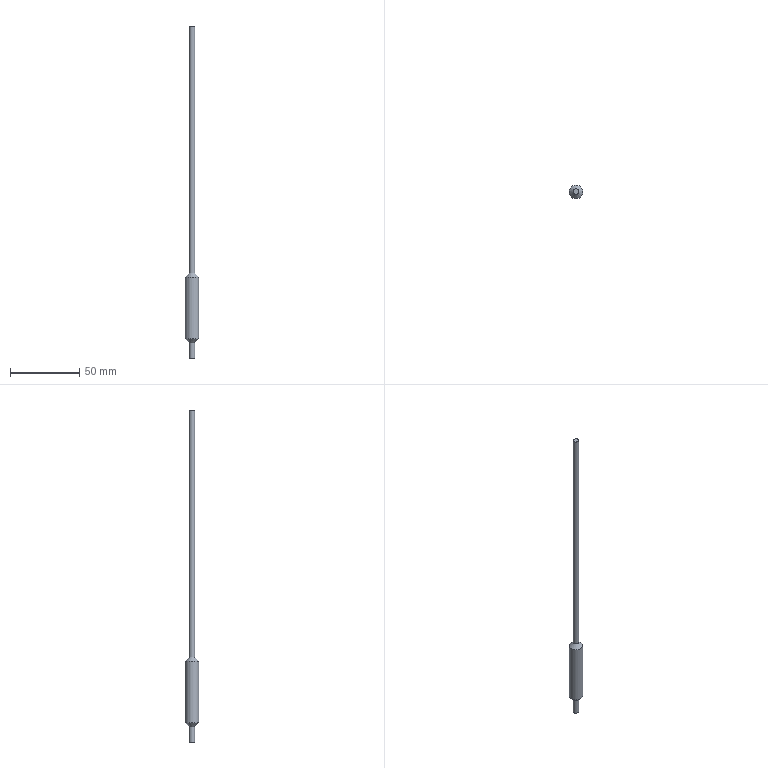Component | NX | MANDREL | 1 solid | 7 faces | box 10 x 10 x 239 mm | volume 6076 mm3 | cylinder 3 | plane 2 | cone 2 | commonest cylinder face diameters 4 x2 10 x1
STEP:
#1=CARTESIAN_POINT('',(0.,0.,0.));
#2=DIRECTION('',(0.,0.,1.));
#3=DIRECTION('',(1.,0.,0.));
#4=AXIS2_PLACEMENT_3D('',#1,#2,#3);
#5=CARTESIAN_POINT('',(-146.777,2.,63.4));
#6=VERTEX_POINT('',#5);
#7=CARTESIAN_POINT('',(-146.777,0.,63.4));
#8=DIRECTION('',(0.,0.,-1.));
#9=DIRECTION('',(0.,1.,0.));
#10=AXIS2_PLACEMENT_3D('',#7,#8,#9);
#11=CIRCLE('',#10,2.);
#12=CARTESIAN_POINT('',(-146.777,0.,63.4));
#13=DIRECTION('',(0.,0.,-1.));
#14=DIRECTION('',(0.,1.,0.));
#15=AXIS2_PLACEMENT_3D('',#12,#13,#14);
#16=PLANE('',#15);
#17=CARTESIAN_POINT('',(0.,0.));
#18=DIRECTION('',(1.,0.));
#19=AXIS2_PLACEMENT_2D('',#17,#18);
#20=CIRCLE('',#19,2.);
#21=(GEOMETRIC_REPRESENTATION_CONTEXT(2)PARAMETRIC_REPRESENTATION_CONTEXT()REPRESENTATION_CONTEXT('',''));
#22=DEFINITIONAL_REPRESENTATION('',(#20),#21);
#23=PCURVE('',#16,#22);
#24=CARTESIAN_POINT('',(-146.777,0.,63.4));
#25=DIRECTION('',(0.,0.,-1.));
#26=DIRECTION('',(0.,1.,0.));
#27=AXIS2_PLACEMENT_3D('',#24,#25,#26);
#28=CYLINDRICAL_SURFACE('',#27,2.);
#29=CARTESIAN_POINT('',(0.,0.));
#30=DIRECTION('',(1.,0.));
#31=VECTOR('',#30,1.);
#32=LINE('',#29,#31);
#33=(GEOMETRIC_REPRESENTATION_CONTEXT(2)PARAMETRIC_REPRESENTATION_CONTEXT()REPRESENTATION_CONTEXT('',''));
#34=DEFINITIONAL_REPRESENTATION('',(#32),#33);
#35=PCURVE('',#28,#34);
#36=SURFACE_CURVE('',#11,(#23,#35),.PCURVE_S1.);
#37=EDGE_CURVE('',#6,#6,#36,.T.);
#38=ORIENTED_EDGE('',*,*,#37,.T.);
#39=EDGE_LOOP('',(#38));
#40=FACE_BOUND('',#39,.T.);
#41=ADVANCED_FACE('',(#40),#16,.T.);
#42=CARTESIAN_POINT('',(-146.777,2.,74.4));
#43=VERTEX_POINT('',#42);
#44=CARTESIAN_POINT('',(-146.777,0.,74.4));
#45=DIRECTION('',(0.,0.,-1.));
#46=DIRECTION('',(0.,1.,0.));
#47=AXIS2_PLACEMENT_3D('',#44,#45,#46);
#48=CIRCLE('',#47,2.);
#49=CARTESIAN_POINT('',(0.,-11.));
#50=DIRECTION('',(1.,0.));
#51=VECTOR('',#50,1.);
#52=LINE('',#49,#51);
#53=(GEOMETRIC_REPRESENTATION_CONTEXT(2)PARAMETRIC_REPRESENTATION_CONTEXT()REPRESENTATION_CONTEXT('',''));
#54=DEFINITIONAL_REPRESENTATION('',(#52),#53);
#55=PCURVE('',#28,#54);
#56=CARTESIAN_POINT('',(-146.777,0.,74.4));
#57=DIRECTION('',(0.,0.,1.));
#58=DIRECTION('',(0.,-1.,0.));
#59=AXIS2_PLACEMENT_3D('',#56,#57,#58);
#60=CONICAL_SURFACE('',#59,2.,0.7854);
#61=CARTESIAN_POINT('',(9.425,0.));
#62=DIRECTION('',(-1.,0.));
#63=VECTOR('',#62,1.);
#64=LINE('',#61,#63);
#65=(GEOMETRIC_REPRESENTATION_CONTEXT(2)PARAMETRIC_REPRESENTATION_CONTEXT()REPRESENTATION_CONTEXT('',''));
#66=DEFINITIONAL_REPRESENTATION('',(#64),#65);
#67=PCURVE('',#60,#66);
#68=SURFACE_CURVE('',#48,(#55,#67),.PCURVE_S1.);
#69=EDGE_CURVE('',#43,#43,#68,.T.);
#70=ORIENTED_EDGE('',*,*,#69,.T.);
#71=CARTESIAN_POINT('',(-146.777,2.,74.4));
#72=CARTESIAN_POINT('',(-146.777,2.,63.4));
#73=B_SPLINE_CURVE_WITH_KNOTS('',1,(#71,#72),.UNSPECIFIED.,.F.,.F.,(2,2),(-11.,0.),.PIECEWISE_BEZIER_KNOTS.);
#74=CARTESIAN_POINT('',(6.283,0.));
#75=DIRECTION('',(0.,1.));
#76=VECTOR('',#75,1.);
#77=LINE('',#74,#76);
#78=(GEOMETRIC_REPRESENTATION_CONTEXT(2)PARAMETRIC_REPRESENTATION_CONTEXT()REPRESENTATION_CONTEXT('',''));
#79=DEFINITIONAL_REPRESENTATION('',(#77),#78);
#80=PCURVE('',#28,#79);
#81=CARTESIAN_POINT('',(0.,0.));
#82=DIRECTION('',(0.,1.));
#83=VECTOR('',#82,1.);
#84=LINE('',#81,#83);
#85=(GEOMETRIC_REPRESENTATION_CONTEXT(2)PARAMETRIC_REPRESENTATION_CONTEXT()REPRESENTATION_CONTEXT('',''));
#86=DEFINITIONAL_REPRESENTATION('',(#84),#85);
#87=PCURVE('',#28,#86);
#88=SEAM_CURVE('',#73,(#80,#87),.PCURVE_S1.);
#89=EDGE_CURVE('',#43,#6,#88,.T.);
#90=ORIENTED_EDGE('',*,*,#89,.T.);
#91=ORIENTED_EDGE('',*,*,#37,.F.);
#92=ORIENTED_EDGE('',*,*,#89,.F.);
#93=EDGE_LOOP('',(#70,#90,#91,#92));
#94=FACE_BOUND('',#93,.T.);
#95=ADVANCED_FACE('',(#94),#28,.T.);
#96=CARTESIAN_POINT('',(-146.777,5.,77.4));
#97=VERTEX_POINT('',#96);
#98=CARTESIAN_POINT('',(-146.777,0.,77.4));
#99=DIRECTION('',(0.,0.,-1.));
#100=DIRECTION('',(0.,1.,0.));
#101=AXIS2_PLACEMENT_3D('',#98,#99,#100);
#102=CIRCLE('',#101,5.);
#103=CARTESIAN_POINT('',(9.425,3.));
#104=DIRECTION('',(-1.,0.));
#105=VECTOR('',#104,1.);
#106=LINE('',#103,#105);
#107=(GEOMETRIC_REPRESENTATION_CONTEXT(2)PARAMETRIC_REPRESENTATION_CONTEXT()REPRESENTATION_CONTEXT('',''));
#108=DEFINITIONAL_REPRESENTATION('',(#106),#107);
#109=PCURVE('',#60,#108);
#110=CARTESIAN_POINT('',(-146.777,0.,63.4));
#111=DIRECTION('',(0.,0.,-1.));
#112=DIRECTION('',(0.,1.,0.));
#113=AXIS2_PLACEMENT_3D('',#110,#111,#112);
#114=CYLINDRICAL_SURFACE('',#113,5.);
#115=CARTESIAN_POINT('',(0.,-14.));
#116=DIRECTION('',(1.,0.));
#117=VECTOR('',#116,1.);
#118=LINE('',#115,#117);
#119=(GEOMETRIC_REPRESENTATION_CONTEXT(2)PARAMETRIC_REPRESENTATION_CONTEXT()REPRESENTATION_CONTEXT('',''));
#120=DEFINITIONAL_REPRESENTATION('',(#118),#119);
#121=PCURVE('',#114,#120);
#122=SURFACE_CURVE('',#102,(#109,#121),.PCURVE_S1.);
#123=EDGE_CURVE('',#97,#97,#122,.T.);
#124=ORIENTED_EDGE('',*,*,#123,.T.);
#125=CARTESIAN_POINT('',(-146.777,2.,74.4));
#126=CARTESIAN_POINT('',(-146.777,5.,77.4));
#127=B_SPLINE_CURVE_WITH_KNOTS('',1,(#125,#126),.UNSPECIFIED.,.F.,.F.,(2,2),(0.,4.243),.PIECEWISE_BEZIER_KNOTS.);
#128=CARTESIAN_POINT('',(3.142,0.));
#129=DIRECTION('',(0.,1.));
#130=VECTOR('',#129,1.);
#131=LINE('',#128,#130);
#132=(GEOMETRIC_REPRESENTATION_CONTEXT(2)PARAMETRIC_REPRESENTATION_CONTEXT()REPRESENTATION_CONTEXT('',''));
#133=DEFINITIONAL_REPRESENTATION('',(#131),#132);
#134=PCURVE('',#60,#133);
#135=CARTESIAN_POINT('',(9.425,0.));
#136=DIRECTION('',(0.,1.));
#137=VECTOR('',#136,1.);
#138=LINE('',#135,#137);
#139=(GEOMETRIC_REPRESENTATION_CONTEXT(2)PARAMETRIC_REPRESENTATION_CONTEXT()REPRESENTATION_CONTEXT('',''));
#140=DEFINITIONAL_REPRESENTATION('',(#138),#139);
#141=PCURVE('',#60,#140);
#142=SEAM_CURVE('',#127,(#134,#141),.PCURVE_S1.);
#143=EDGE_CURVE('',#43,#97,#142,.T.);
#144=ORIENTED_EDGE('',*,*,#143,.F.);
#145=ORIENTED_EDGE('',*,*,#69,.F.);
#146=ORIENTED_EDGE('',*,*,#143,.T.);
#147=EDGE_LOOP('',(#124,#144,#145,#146));
#148=FACE_BOUND('',#147,.T.);
#149=ADVANCED_FACE('',(#148),#60,.T.);
#150=CARTESIAN_POINT('',(-146.777,5.,121.4));
#151=VERTEX_POINT('',#150);
#152=CARTESIAN_POINT('',(-146.777,0.,121.4));
#153=DIRECTION('',(0.,0.,-1.));
#154=DIRECTION('',(0.,1.,0.));
#155=AXIS2_PLACEMENT_3D('',#152,#153,#154);
#156=CIRCLE('',#155,5.);
#157=CARTESIAN_POINT('',(0.,-58.));
#158=DIRECTION('',(1.,0.));
#159=VECTOR('',#158,1.);
#160=LINE('',#157,#159);
#161=(GEOMETRIC_REPRESENTATION_CONTEXT(2)PARAMETRIC_REPRESENTATION_CONTEXT()REPRESENTATION_CONTEXT('',''));
#162=DEFINITIONAL_REPRESENTATION('',(#160),#161);
#163=PCURVE('',#114,#162);
#164=CARTESIAN_POINT('',(-146.777,0.,121.4));
#165=DIRECTION('',(0.,0.,-1.));
#166=DIRECTION('',(0.,1.,0.));
#167=AXIS2_PLACEMENT_3D('',#164,#165,#166);
#168=CONICAL_SURFACE('',#167,5.,0.7854);
#169=CARTESIAN_POINT('',(0.,0.));
#170=DIRECTION('',(1.,0.));
#171=VECTOR('',#170,1.);
#172=LINE('',#169,#171);
#173=(GEOMETRIC_REPRESENTATION_CONTEXT(2)PARAMETRIC_REPRESENTATION_CONTEXT()REPRESENTATION_CONTEXT('',''));
#174=DEFINITIONAL_REPRESENTATION('',(#172),#173);
#175=PCURVE('',#168,#174);
#176=SURFACE_CURVE('',#156,(#163,#175),.PCURVE_S1.);
#177=EDGE_CURVE('',#151,#151,#176,.T.);
#178=ORIENTED_EDGE('',*,*,#177,.T.);
#179=CARTESIAN_POINT('',(-146.777,5.,121.4));
#180=CARTESIAN_POINT('',(-146.777,5.,77.4));
#181=B_SPLINE_CURVE_WITH_KNOTS('',1,(#179,#180),.UNSPECIFIED.,.F.,.F.,(2,2),(-58.,-14.),.PIECEWISE_BEZIER_KNOTS.);
#182=CARTESIAN_POINT('',(6.283,0.));
#183=DIRECTION('',(0.,1.));
#184=VECTOR('',#183,1.);
#185=LINE('',#182,#184);
#186=(GEOMETRIC_REPRESENTATION_CONTEXT(2)PARAMETRIC_REPRESENTATION_CONTEXT()REPRESENTATION_CONTEXT('',''));
#187=DEFINITIONAL_REPRESENTATION('',(#185),#186);
#188=PCURVE('',#114,#187);
#189=CARTESIAN_POINT('',(0.,0.));
#190=DIRECTION('',(0.,1.));
#191=VECTOR('',#190,1.);
#192=LINE('',#189,#191);
#193=(GEOMETRIC_REPRESENTATION_CONTEXT(2)PARAMETRIC_REPRESENTATION_CONTEXT()REPRESENTATION_CONTEXT('',''));
#194=DEFINITIONAL_REPRESENTATION('',(#192),#193);
#195=PCURVE('',#114,#194);
#196=SEAM_CURVE('',#181,(#188,#195),.PCURVE_S1.);
#197=EDGE_CURVE('',#151,#97,#196,.T.);
#198=ORIENTED_EDGE('',*,*,#197,.T.);
#199=ORIENTED_EDGE('',*,*,#123,.F.);
#200=ORIENTED_EDGE('',*,*,#197,.F.);
#201=EDGE_LOOP('',(#178,#198,#199,#200));
#202=FACE_BOUND('',#201,.T.);
#203=ADVANCED_FACE('',(#202),#114,.T.);
#204=CARTESIAN_POINT('',(-146.777,2.,124.4));
#205=VERTEX_POINT('',#204);
#206=CARTESIAN_POINT('',(-146.777,0.,124.4));
#207=DIRECTION('',(0.,0.,-1.));
#208=DIRECTION('',(0.,1.,0.));
#209=AXIS2_PLACEMENT_3D('',#206,#207,#208);
#210=CIRCLE('',#209,2.);
#211=CARTESIAN_POINT('',(0.,-3.));
#212=DIRECTION('',(1.,0.));
#213=VECTOR('',#212,1.);
#214=LINE('',#211,#213);
#215=(GEOMETRIC_REPRESENTATION_CONTEXT(2)PARAMETRIC_REPRESENTATION_CONTEXT()REPRESENTATION_CONTEXT('',''));
#216=DEFINITIONAL_REPRESENTATION('',(#214),#215);
#217=PCURVE('',#168,#216);
#218=CARTESIAN_POINT('',(-146.777,0.,63.4));
#219=DIRECTION('',(0.,0.,-1.));
#220=DIRECTION('',(0.,1.,0.));
#221=AXIS2_PLACEMENT_3D('',#218,#219,#220);
#222=CYLINDRICAL_SURFACE('',#221,2.);
#223=CARTESIAN_POINT('',(0.,-61.));
#224=DIRECTION('',(1.,0.));
#225=VECTOR('',#224,1.);
#226=LINE('',#223,#225);
#227=(GEOMETRIC_REPRESENTATION_CONTEXT(2)PARAMETRIC_REPRESENTATION_CONTEXT()REPRESENTATION_CONTEXT('',''));
#228=DEFINITIONAL_REPRESENTATION('',(#226),#227);
#229=PCURVE('',#222,#228);
#230=SURFACE_CURVE('',#210,(#217,#229),.PCURVE_S1.);
#231=EDGE_CURVE('',#205,#205,#230,.T.);
#232=ORIENTED_EDGE('',*,*,#231,.T.);
#233=CARTESIAN_POINT('',(-146.777,2.,124.4));
#234=CARTESIAN_POINT('',(-146.777,5.,121.4));
#235=B_SPLINE_CURVE_WITH_KNOTS('',1,(#233,#234),.UNSPECIFIED.,.F.,.F.,(2,2),(-4.243,0.),.PIECEWISE_BEZIER_KNOTS.);
#236=CARTESIAN_POINT('',(6.283,0.));
#237=DIRECTION('',(0.,1.));
#238=VECTOR('',#237,1.);
#239=LINE('',#236,#238);
#240=(GEOMETRIC_REPRESENTATION_CONTEXT(2)PARAMETRIC_REPRESENTATION_CONTEXT()REPRESENTATION_CONTEXT('',''));
#241=DEFINITIONAL_REPRESENTATION('',(#239),#240);
#242=PCURVE('',#168,#241);
#243=CARTESIAN_POINT('',(0.,0.));
#244=DIRECTION('',(0.,1.));
#245=VECTOR('',#244,1.);
#246=LINE('',#243,#245);
#247=(GEOMETRIC_REPRESENTATION_CONTEXT(2)PARAMETRIC_REPRESENTATION_CONTEXT()REPRESENTATION_CONTEXT('',''));
#248=DEFINITIONAL_REPRESENTATION('',(#246),#247);
#249=PCURVE('',#168,#248);
#250=SEAM_CURVE('',#235,(#242,#249),.PCURVE_S1.);
#251=EDGE_CURVE('',#205,#151,#250,.T.);
#252=ORIENTED_EDGE('',*,*,#251,.T.);
#253=ORIENTED_EDGE('',*,*,#177,.F.);
#254=ORIENTED_EDGE('',*,*,#251,.F.);
#255=EDGE_LOOP('',(#232,#252,#253,#254));
#256=FACE_BOUND('',#255,.T.);
#257=ADVANCED_FACE('',(#256),#168,.T.);
#258=CARTESIAN_POINT('',(-146.777,2.,302.4));
#259=VERTEX_POINT('',#258);
#260=CARTESIAN_POINT('',(-146.777,0.,302.4));
#261=DIRECTION('',(0.,0.,-1.));
#262=DIRECTION('',(0.,1.,0.));
#263=AXIS2_PLACEMENT_3D('',#260,#261,#262);
#264=CIRCLE('',#263,2.);
#265=CARTESIAN_POINT('',(0.,-239.));
#266=DIRECTION('',(1.,0.));
#267=VECTOR('',#266,1.);
#268=LINE('',#265,#267);
#269=(GEOMETRIC_REPRESENTATION_CONTEXT(2)PARAMETRIC_REPRESENTATION_CONTEXT()REPRESENTATION_CONTEXT('',''));
#270=DEFINITIONAL_REPRESENTATION('',(#268),#269);
#271=PCURVE('',#222,#270);
#272=CARTESIAN_POINT('',(-144.777,0.,302.4));
#273=DIRECTION('',(0.,0.,1.));
#274=DIRECTION('',(0.,-1.,0.));
#275=AXIS2_PLACEMENT_3D('',#272,#273,#274);
#276=PLANE('',#275);
#277=CARTESIAN_POINT('',(-2.,-2.));
#278=CARTESIAN_POINT('',(-2.,1.464));
#279=CARTESIAN_POINT('',(1.,-0.2679));
#280=CARTESIAN_POINT('',(4.,-2.));
#281=CARTESIAN_POINT('',(1.,-3.732));
#282=CARTESIAN_POINT('',(-2.,-5.464));
#283=CARTESIAN_POINT('',(-2.,-2.));
#284=(BOUNDED_CURVE()B_SPLINE_CURVE(2,(#277,#278,#279,#280,#281,#282,#283),.UNSPECIFIED.,.T.,.F.)B_SPLINE_CURVE_WITH_KNOTS((1,2,2,2,2,1),(-2.094,0.,2.094,4.189,6.283,8.378),.UNSPECIFIED.)CURVE()GEOMETRIC_REPRESENTATION_ITEM()RATIONAL_B_SPLINE_CURVE((1.,0.5,1.,0.5,1.,0.5,1.))REPRESENTATION_ITEM(''));
#285=(GEOMETRIC_REPRESENTATION_CONTEXT(2)PARAMETRIC_REPRESENTATION_CONTEXT()REPRESENTATION_CONTEXT('',''));
#286=DEFINITIONAL_REPRESENTATION('',(#284),#285);
#287=PCURVE('',#276,#286);
#288=SURFACE_CURVE('',#264,(#271,#287),.PCURVE_S1.);
#289=EDGE_CURVE('',#259,#259,#288,.T.);
#290=ORIENTED_EDGE('',*,*,#289,.T.);
#291=CARTESIAN_POINT('',(-146.777,2.,302.4));
#292=CARTESIAN_POINT('',(-146.777,2.,124.4));
#293=B_SPLINE_CURVE_WITH_KNOTS('',1,(#291,#292),.UNSPECIFIED.,.F.,.F.,(2,2),(-239.,-61.),.PIECEWISE_BEZIER_KNOTS.);
#294=CARTESIAN_POINT('',(6.283,0.));
#295=DIRECTION('',(0.,1.));
#296=VECTOR('',#295,1.);
#297=LINE('',#294,#296);
#298=(GEOMETRIC_REPRESENTATION_CONTEXT(2)PARAMETRIC_REPRESENTATION_CONTEXT()REPRESENTATION_CONTEXT('',''));
#299=DEFINITIONAL_REPRESENTATION('',(#297),#298);
#300=PCURVE('',#222,#299);
#301=CARTESIAN_POINT('',(0.,0.));
#302=DIRECTION('',(0.,1.));
#303=VECTOR('',#302,1.);
#304=LINE('',#301,#303);
#305=(GEOMETRIC_REPRESENTATION_CONTEXT(2)PARAMETRIC_REPRESENTATION_CONTEXT()REPRESENTATION_CONTEXT('',''));
#306=DEFINITIONAL_REPRESENTATION('',(#304),#305);
#307=PCURVE('',#222,#306);
#308=SEAM_CURVE('',#293,(#300,#307),.PCURVE_S1.);
#309=EDGE_CURVE('',#259,#205,#308,.T.);
#310=ORIENTED_EDGE('',*,*,#309,.T.);
#311=ORIENTED_EDGE('',*,*,#231,.F.);
#312=ORIENTED_EDGE('',*,*,#309,.F.);
#313=EDGE_LOOP('',(#290,#310,#311,#312));
#314=FACE_BOUND('',#313,.T.);
#315=ADVANCED_FACE('',(#314),#222,.T.);
#316=ORIENTED_EDGE('',*,*,#289,.F.);
#317=EDGE_LOOP('',(#316));
#318=FACE_BOUND('',#317,.T.);
#319=ADVANCED_FACE('',(#318),#276,.T.);
#320=CLOSED_SHELL('',(#41,#95,#149,#203,#257,#315,#319));
#321=MANIFOLD_SOLID_BREP('',#320);
#322=(LENGTH_UNIT()NAMED_UNIT(*)SI_UNIT(.MILLI.,.METRE.));
#323=UNCERTAINTY_MEASURE_WITH_UNIT(LENGTH_MEASURE(0.00001),#322,'','');
#324=(NAMED_UNIT(*)PLANE_ANGLE_UNIT()SI_UNIT($,.RADIAN.));
#325=(NAMED_UNIT(*)SI_UNIT($,.STERADIAN.)SOLID_ANGLE_UNIT());
#326=(GEOMETRIC_REPRESENTATION_CONTEXT(3)GLOBAL_UNCERTAINTY_ASSIGNED_CONTEXT((#323))GLOBAL_UNIT_ASSIGNED_CONTEXT((#322,#324,#325))REPRESENTATION_CONTEXT('',''));
#327=ADVANCED_BREP_SHAPE_REPRESENTATION('',(#4,#321),#326);